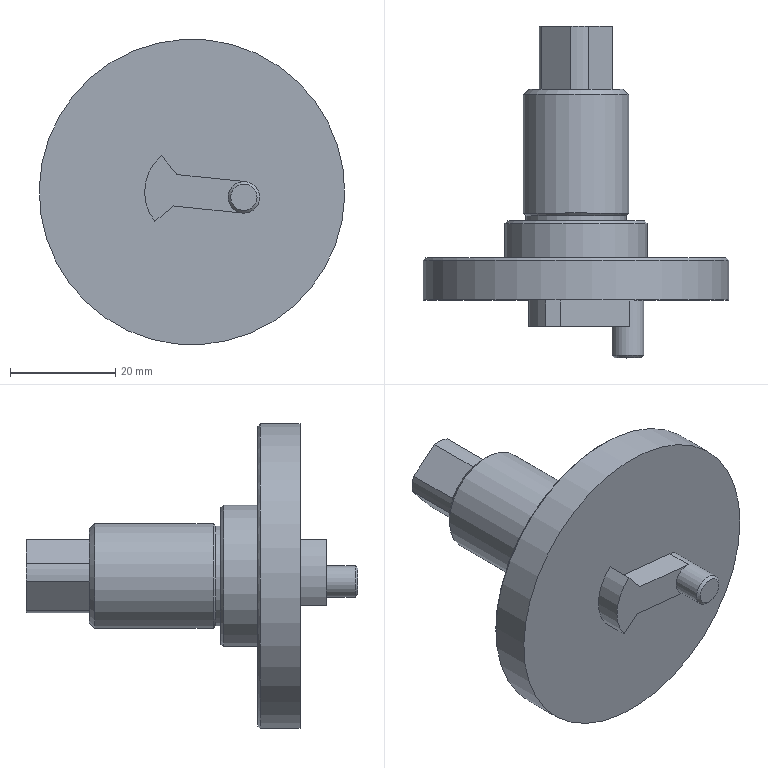Component | NX | INDEXING_SHAFT | 1 solid | 30 faces | volume 35401 mm3 | plane 15 | cylinder 10 | cone 5 | commonest cylinder face diameters 14 x4 20 x1 19 x1 27 x1 58 x1 18 x1 6 x1